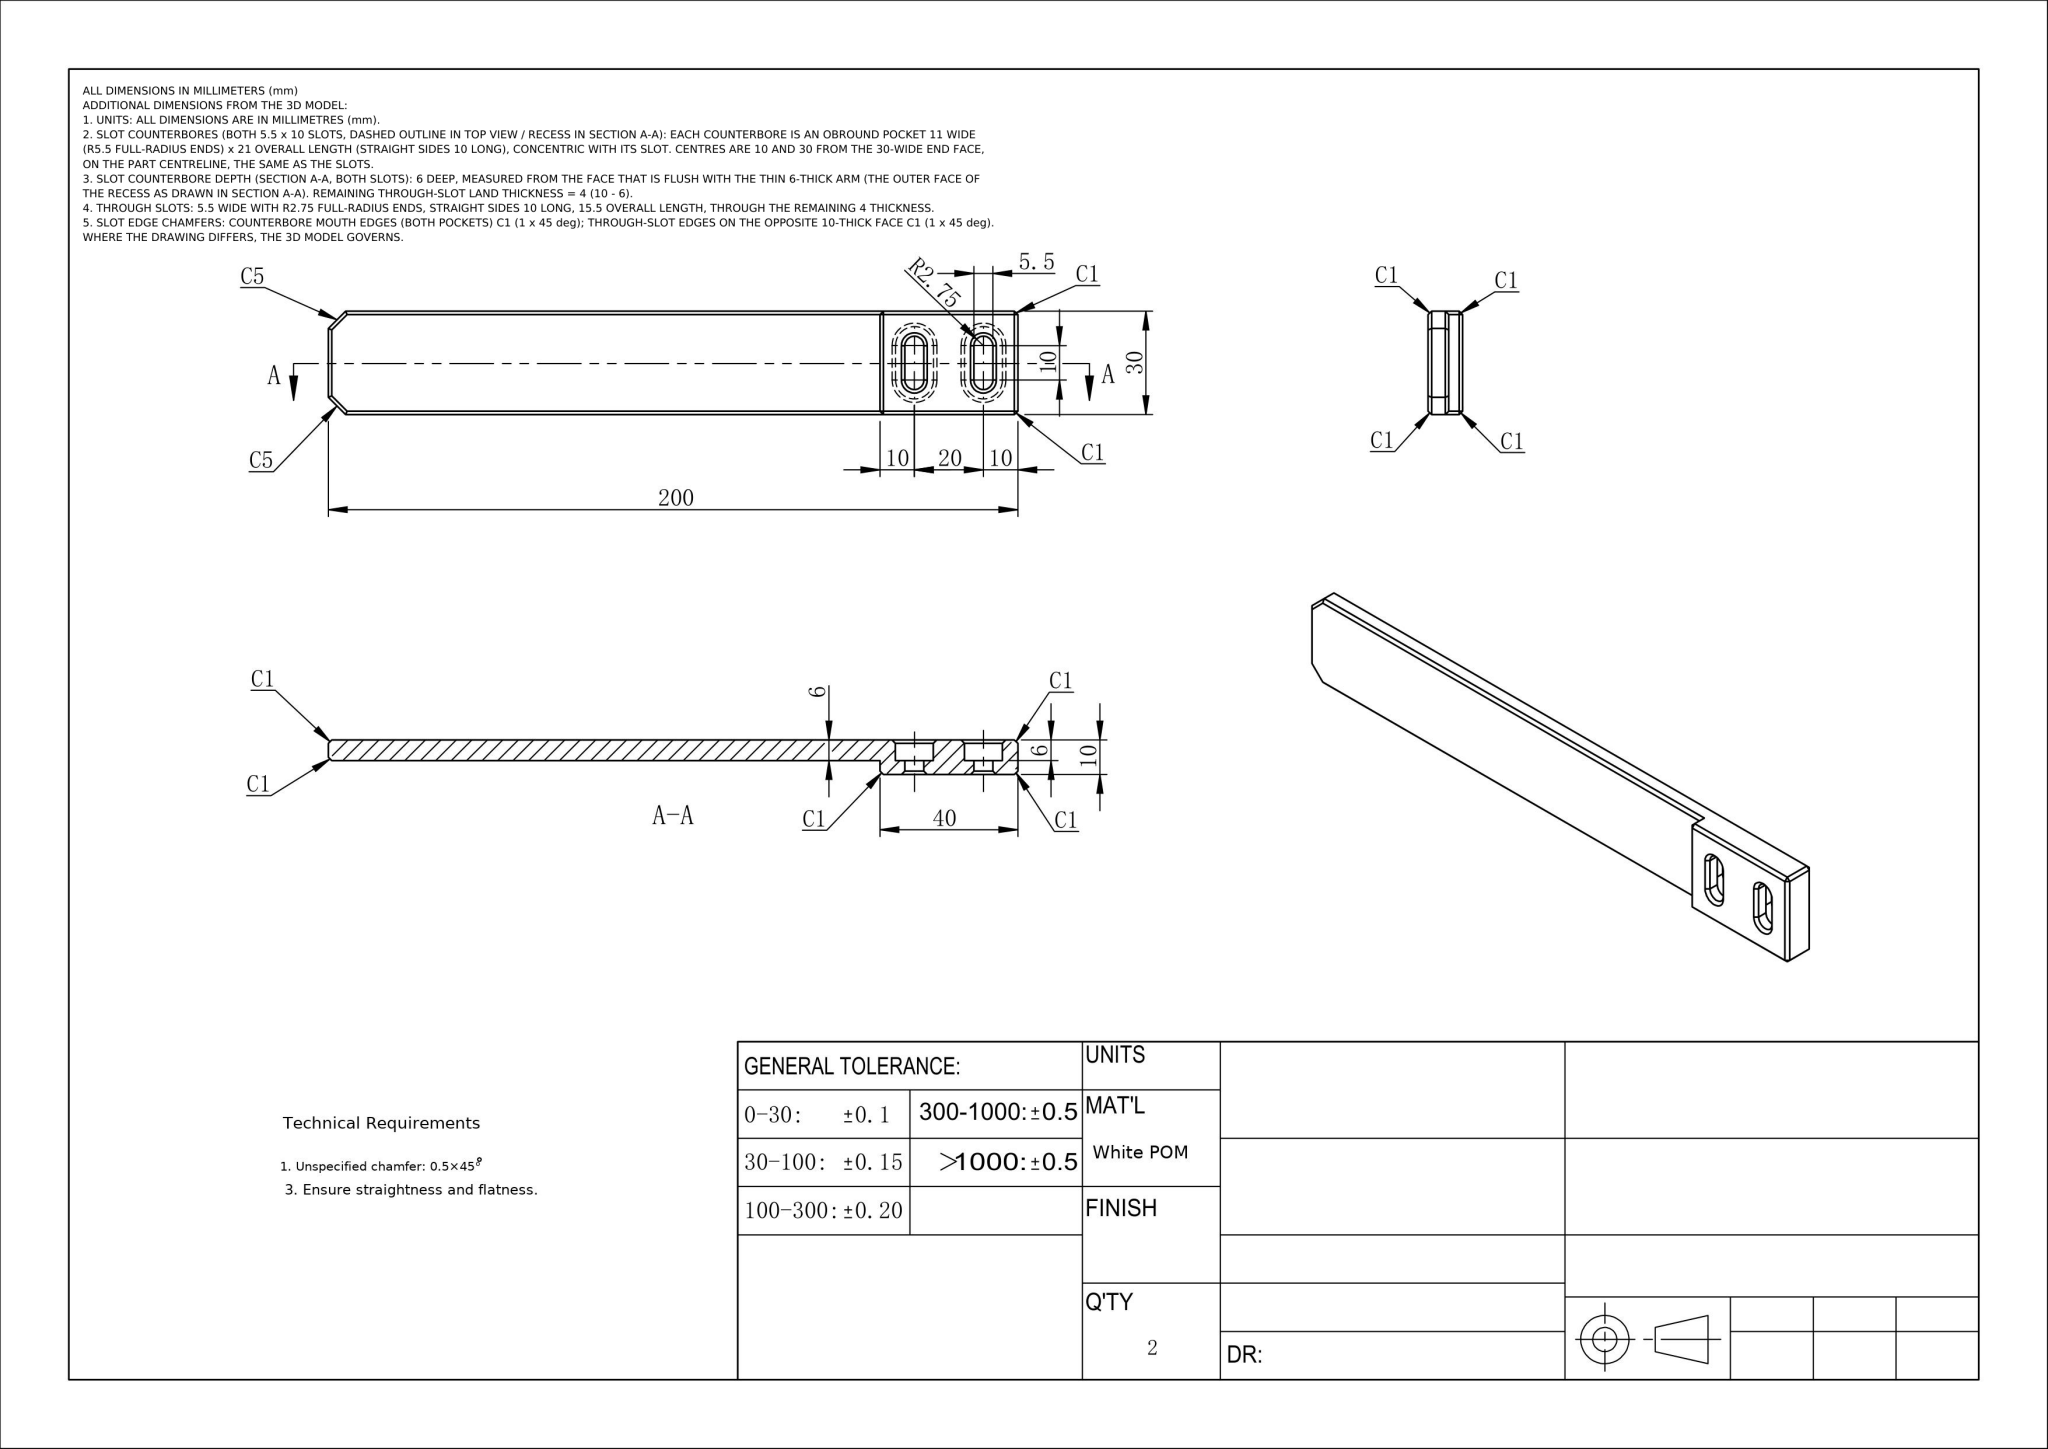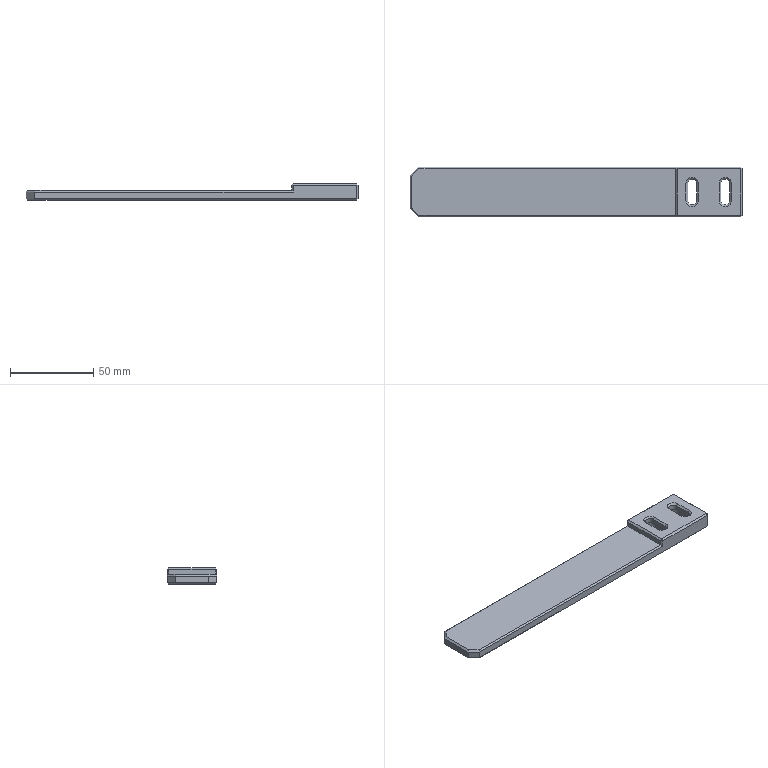Part | NX | mm | Stepped Dual-Slot Mounting Bar | 1 solid | 69 faces | box 200 x 30 x 10 mm | volume 36985 mm3 | plane 53 | cylinder 8 | cone 8 | commonest cylinder face diameters 5.5 x4 11 x4